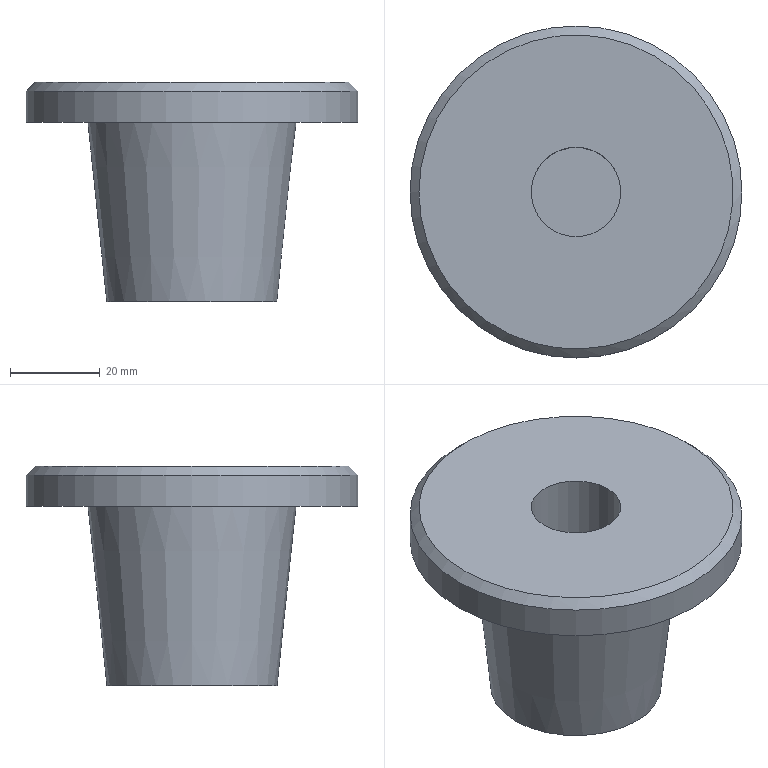Component | NX | CH3404_19_3-6 | 1 solid | 8 faces | box 74 x 74 x 49 mm | volume 82142 mm3 | plane 4 | cylinder 2 | cone 2 | commonest cylinder face diameters 74 x1 20 x1
STEP:
#1=CARTESIAN_POINT('',(0.,0.,0.));
#2=DIRECTION('',(0.,0.,1.));
#3=DIRECTION('',(1.,0.,0.));
#4=AXIS2_PLACEMENT_3D('',#1,#2,#3);
#5=CARTESIAN_POINT('',(-37.,0.,96.55));
#6=VERTEX_POINT('',#5);
#7=CARTESIAN_POINT('',(0.,0.,96.55));
#8=DIRECTION('',(0.,0.,-1.));
#9=DIRECTION('',(-1.,0.,0.));
#10=AXIS2_PLACEMENT_3D('',#7,#8,#9);
#11=CIRCLE('',#10,37.);
#12=CARTESIAN_POINT('',(0.,0.,56.55));
#13=DIRECTION('',(0.,0.,-1.));
#14=DIRECTION('',(-1.,0.,0.));
#15=AXIS2_PLACEMENT_3D('',#12,#13,#14);
#16=CYLINDRICAL_SURFACE('',#15,37.);
#17=CARTESIAN_POINT('',(0.,-40.));
#18=DIRECTION('',(1.,0.));
#19=VECTOR('',#18,1.);
#20=LINE('',#17,#19);
#21=(GEOMETRIC_REPRESENTATION_CONTEXT(2)PARAMETRIC_REPRESENTATION_CONTEXT()REPRESENTATION_CONTEXT('',''));
#22=DEFINITIONAL_REPRESENTATION('',(#20),#21);
#23=PCURVE('',#16,#22);
#24=CARTESIAN_POINT('',(0.,-37.,96.55));
#25=DIRECTION('',(0.,0.,1.));
#26=DIRECTION('',(1.,0.,0.));
#27=AXIS2_PLACEMENT_3D('',#24,#25,#26);
#28=PLANE('',#27);
#29=CARTESIAN_POINT('',(-37.,37.));
#30=CARTESIAN_POINT('',(-37.,101.086));
#31=CARTESIAN_POINT('',(18.5,69.043));
#32=CARTESIAN_POINT('',(74.,37.));
#33=CARTESIAN_POINT('',(18.5,4.957));
#34=CARTESIAN_POINT('',(-37.,-27.086));
#35=CARTESIAN_POINT('',(-37.,37.));
#36=(BOUNDED_CURVE()B_SPLINE_CURVE(2,(#29,#30,#31,#32,#33,#34,#35),.UNSPECIFIED.,.T.,.F.)B_SPLINE_CURVE_WITH_KNOTS((1,2,2,2,2,1),(-2.094,0.,2.094,4.189,6.283,8.378),.UNSPECIFIED.)CURVE()GEOMETRIC_REPRESENTATION_ITEM()RATIONAL_B_SPLINE_CURVE((1.,0.5,1.,0.5,1.,0.5,1.))REPRESENTATION_ITEM(''));
#37=(GEOMETRIC_REPRESENTATION_CONTEXT(2)PARAMETRIC_REPRESENTATION_CONTEXT()REPRESENTATION_CONTEXT('',''));
#38=DEFINITIONAL_REPRESENTATION('',(#36),#37);
#39=PCURVE('',#28,#38);
#40=SURFACE_CURVE('',#11,(#23,#39),.PCURVE_S1.);
#41=EDGE_CURVE('',#6,#6,#40,.T.);
#42=ORIENTED_EDGE('',*,*,#41,.F.);
#43=CARTESIAN_POINT('',(-37.,0.,103.55));
#44=VERTEX_POINT('',#43);
#45=CARTESIAN_POINT('',(-37.,-0.,103.55));
#46=CARTESIAN_POINT('',(-37.,-0.,96.55));
#47=B_SPLINE_CURVE_WITH_KNOTS('',1,(#45,#46),.UNSPECIFIED.,.F.,.F.,(2,2),(-47.,-40.),.PIECEWISE_BEZIER_KNOTS.);
#48=CARTESIAN_POINT('',(0.,0.));
#49=DIRECTION('',(0.,1.));
#50=VECTOR('',#49,1.);
#51=LINE('',#48,#50);
#52=(GEOMETRIC_REPRESENTATION_CONTEXT(2)PARAMETRIC_REPRESENTATION_CONTEXT()REPRESENTATION_CONTEXT('',''));
#53=DEFINITIONAL_REPRESENTATION('',(#51),#52);
#54=PCURVE('',#16,#53);
#55=CARTESIAN_POINT('',(6.283,0.));
#56=DIRECTION('',(0.,1.));
#57=VECTOR('',#56,1.);
#58=LINE('',#55,#57);
#59=(GEOMETRIC_REPRESENTATION_CONTEXT(2)PARAMETRIC_REPRESENTATION_CONTEXT()REPRESENTATION_CONTEXT('',''));
#60=DEFINITIONAL_REPRESENTATION('',(#58),#59);
#61=PCURVE('',#16,#60);
#62=SEAM_CURVE('',#47,(#54,#61),.PCURVE_S1.);
#63=EDGE_CURVE('',#44,#6,#62,.T.);
#64=ORIENTED_EDGE('',*,*,#63,.F.);
#65=CARTESIAN_POINT('',(0.,0.,103.55));
#66=DIRECTION('',(0.,0.,-1.));
#67=DIRECTION('',(-1.,0.,0.));
#68=AXIS2_PLACEMENT_3D('',#65,#66,#67);
#69=CIRCLE('',#68,37.);
#70=CARTESIAN_POINT('',(0.,-47.));
#71=DIRECTION('',(1.,0.));
#72=VECTOR('',#71,1.);
#73=LINE('',#70,#72);
#74=(GEOMETRIC_REPRESENTATION_CONTEXT(2)PARAMETRIC_REPRESENTATION_CONTEXT()REPRESENTATION_CONTEXT('',''));
#75=DEFINITIONAL_REPRESENTATION('',(#73),#74);
#76=PCURVE('',#16,#75);
#77=CARTESIAN_POINT('',(0.,0.,105.55));
#78=DIRECTION('',(0.,0.,-1.));
#79=DIRECTION('',(-1.,0.,0.));
#80=AXIS2_PLACEMENT_3D('',#77,#78,#79);
#81=CONICAL_SURFACE('',#80,35.,0.7854);
#82=CARTESIAN_POINT('',(0.,2.));
#83=DIRECTION('',(1.,0.));
#84=VECTOR('',#83,1.);
#85=LINE('',#82,#84);
#86=(GEOMETRIC_REPRESENTATION_CONTEXT(2)PARAMETRIC_REPRESENTATION_CONTEXT()REPRESENTATION_CONTEXT('',''));
#87=DEFINITIONAL_REPRESENTATION('',(#85),#86);
#88=PCURVE('',#81,#87);
#89=SURFACE_CURVE('',#69,(#76,#88),.PCURVE_S1.);
#90=EDGE_CURVE('',#44,#44,#89,.T.);
#91=ORIENTED_EDGE('',*,*,#90,.T.);
#92=ORIENTED_EDGE('',*,*,#63,.T.);
#93=EDGE_LOOP('',(#42,#64,#91,#92));
#94=FACE_BOUND('',#93,.T.);
#95=ADVANCED_FACE('',(#94),#16,.T.);
#96=CARTESIAN_POINT('',(-23.204,0.,96.55));
#97=VERTEX_POINT('',#96);
#98=CARTESIAN_POINT('',(0.,0.,96.55));
#99=DIRECTION('',(0.,0.,-1.));
#100=DIRECTION('',(-1.,0.,0.));
#101=AXIS2_PLACEMENT_3D('',#98,#99,#100);
#102=CIRCLE('',#101,23.204);
#103=CARTESIAN_POINT('',(-23.204,37.));
#104=CARTESIAN_POINT('',(-23.204,77.191));
#105=CARTESIAN_POINT('',(11.602,57.095));
#106=CARTESIAN_POINT('',(46.408,37.));
#107=CARTESIAN_POINT('',(11.602,16.905));
#108=CARTESIAN_POINT('',(-23.204,-3.191));
#109=CARTESIAN_POINT('',(-23.204,37.));
#110=(BOUNDED_CURVE()B_SPLINE_CURVE(2,(#103,#104,#105,#106,#107,#108,#109),.UNSPECIFIED.,.T.,.F.)B_SPLINE_CURVE_WITH_KNOTS((1,2,2,2,2,1),(-2.094,0.,2.094,4.189,6.283,8.378),.UNSPECIFIED.)CURVE()GEOMETRIC_REPRESENTATION_ITEM()RATIONAL_B_SPLINE_CURVE((1.,0.5,1.,0.5,1.,0.5,1.))REPRESENTATION_ITEM(''));
#111=(GEOMETRIC_REPRESENTATION_CONTEXT(2)PARAMETRIC_REPRESENTATION_CONTEXT()REPRESENTATION_CONTEXT('',''));
#112=DEFINITIONAL_REPRESENTATION('',(#110),#111);
#113=PCURVE('',#28,#112);
#114=CARTESIAN_POINT('',(0.,0.,96.55));
#115=DIRECTION('',(0.,0.,1.));
#116=DIRECTION('',(1.,0.,0.));
#117=AXIS2_PLACEMENT_3D('',#114,#115,#116);
#118=CONICAL_SURFACE('',#117,23.204,0.1047);
#119=CARTESIAN_POINT('',(9.425,0.));
#120=DIRECTION('',(-1.,0.));
#121=VECTOR('',#120,1.);
#122=LINE('',#119,#121);
#123=(GEOMETRIC_REPRESENTATION_CONTEXT(2)PARAMETRIC_REPRESENTATION_CONTEXT()REPRESENTATION_CONTEXT('',''));
#124=DEFINITIONAL_REPRESENTATION('',(#122),#123);
#125=PCURVE('',#118,#124);
#126=SURFACE_CURVE('',#102,(#113,#125),.PCURVE_S1.);
#127=EDGE_CURVE('',#97,#97,#126,.T.);
#128=ORIENTED_EDGE('',*,*,#127,.F.);
#129=EDGE_LOOP('',(#128));
#130=FACE_BOUND('',#129,.T.);
#131=ORIENTED_EDGE('',*,*,#41,.T.);
#132=EDGE_LOOP('',(#131));
#133=FACE_BOUND('',#132,.T.);
#134=ADVANCED_FACE('',(#130,#133),#28,.F.);
#135=CARTESIAN_POINT('',(-19.,0.,56.55));
#136=VERTEX_POINT('',#135);
#137=CARTESIAN_POINT('',(0.,0.,56.55));
#138=DIRECTION('',(0.,0.,-1.));
#139=DIRECTION('',(-1.,0.,0.));
#140=AXIS2_PLACEMENT_3D('',#137,#138,#139);
#141=CIRCLE('',#140,19.);
#142=CARTESIAN_POINT('',(9.425,-40.));
#143=DIRECTION('',(-1.,0.));
#144=VECTOR('',#143,1.);
#145=LINE('',#142,#144);
#146=(GEOMETRIC_REPRESENTATION_CONTEXT(2)PARAMETRIC_REPRESENTATION_CONTEXT()REPRESENTATION_CONTEXT('',''));
#147=DEFINITIONAL_REPRESENTATION('',(#145),#146);
#148=PCURVE('',#118,#147);
#149=CARTESIAN_POINT('',(0.,-19.,56.55));
#150=DIRECTION('',(0.,0.,1.));
#151=DIRECTION('',(1.,0.,0.));
#152=AXIS2_PLACEMENT_3D('',#149,#150,#151);
#153=PLANE('',#152);
#154=CARTESIAN_POINT('',(-19.,19.));
#155=CARTESIAN_POINT('',(-19.,51.909));
#156=CARTESIAN_POINT('',(9.5,35.454));
#157=CARTESIAN_POINT('',(38.,19.));
#158=CARTESIAN_POINT('',(9.5,2.546));
#159=CARTESIAN_POINT('',(-19.,-13.909));
#160=CARTESIAN_POINT('',(-19.,19.));
#161=(BOUNDED_CURVE()B_SPLINE_CURVE(2,(#154,#155,#156,#157,#158,#159,#160),.UNSPECIFIED.,.T.,.F.)B_SPLINE_CURVE_WITH_KNOTS((1,2,2,2,2,1),(-2.094,0.,2.094,4.189,6.283,8.378),.UNSPECIFIED.)CURVE()GEOMETRIC_REPRESENTATION_ITEM()RATIONAL_B_SPLINE_CURVE((1.,0.5,1.,0.5,1.,0.5,1.))REPRESENTATION_ITEM(''));
#162=(GEOMETRIC_REPRESENTATION_CONTEXT(2)PARAMETRIC_REPRESENTATION_CONTEXT()REPRESENTATION_CONTEXT('',''));
#163=DEFINITIONAL_REPRESENTATION('',(#161),#162);
#164=PCURVE('',#153,#163);
#165=SURFACE_CURVE('',#141,(#148,#164),.PCURVE_S1.);
#166=EDGE_CURVE('',#136,#136,#165,.T.);
#167=ORIENTED_EDGE('',*,*,#166,.F.);
#168=CARTESIAN_POINT('',(-19.,0.,56.55));
#169=CARTESIAN_POINT('',(-23.204,0.,96.55));
#170=B_SPLINE_CURVE_WITH_KNOTS('',1,(#168,#169),.UNSPECIFIED.,.F.,.F.,(2,2),(-40.22,0.),.PIECEWISE_BEZIER_KNOTS.);
#171=CARTESIAN_POINT('',(9.425,0.));
#172=DIRECTION('',(0.,1.));
#173=VECTOR('',#172,1.);
#174=LINE('',#171,#173);
#175=(GEOMETRIC_REPRESENTATION_CONTEXT(2)PARAMETRIC_REPRESENTATION_CONTEXT()REPRESENTATION_CONTEXT('',''));
#176=DEFINITIONAL_REPRESENTATION('',(#174),#175);
#177=PCURVE('',#118,#176);
#178=CARTESIAN_POINT('',(3.142,0.));
#179=DIRECTION('',(0.,1.));
#180=VECTOR('',#179,1.);
#181=LINE('',#178,#180);
#182=(GEOMETRIC_REPRESENTATION_CONTEXT(2)PARAMETRIC_REPRESENTATION_CONTEXT()REPRESENTATION_CONTEXT('',''));
#183=DEFINITIONAL_REPRESENTATION('',(#181),#182);
#184=PCURVE('',#118,#183);
#185=SEAM_CURVE('',#170,(#177,#184),.PCURVE_S1.);
#186=EDGE_CURVE('',#136,#97,#185,.T.);
#187=ORIENTED_EDGE('',*,*,#186,.T.);
#188=ORIENTED_EDGE('',*,*,#127,.T.);
#189=ORIENTED_EDGE('',*,*,#186,.F.);
#190=EDGE_LOOP('',(#167,#187,#188,#189));
#191=FACE_BOUND('',#190,.T.);
#192=ADVANCED_FACE('',(#191),#118,.T.);
#193=ORIENTED_EDGE('',*,*,#166,.T.);
#194=EDGE_LOOP('',(#193));
#195=FACE_BOUND('',#194,.T.);
#196=ADVANCED_FACE('',(#195),#153,.F.);
#197=CARTESIAN_POINT('',(-10.,0.,66.55));
#198=VERTEX_POINT('',#197);
#199=CARTESIAN_POINT('',(0.,0.,66.55));
#200=DIRECTION('',(0.,0.,-1.));
#201=DIRECTION('',(-1.,0.,0.));
#202=AXIS2_PLACEMENT_3D('',#199,#200,#201);
#203=CIRCLE('',#202,10.);
#204=CARTESIAN_POINT('',(0.,0.,66.55));
#205=DIRECTION('',(0.,0.,-1.));
#206=DIRECTION('',(-1.,0.,0.));
#207=AXIS2_PLACEMENT_3D('',#204,#205,#206);
#208=PLANE('',#207);
#209=CARTESIAN_POINT('',(0.,0.));
#210=DIRECTION('',(1.,0.));
#211=AXIS2_PLACEMENT_2D('',#209,#210);
#212=CIRCLE('',#211,10.);
#213=(GEOMETRIC_REPRESENTATION_CONTEXT(2)PARAMETRIC_REPRESENTATION_CONTEXT()REPRESENTATION_CONTEXT('',''));
#214=DEFINITIONAL_REPRESENTATION('',(#212),#213);
#215=PCURVE('',#208,#214);
#216=CARTESIAN_POINT('',(0.,0.,56.55));
#217=DIRECTION('',(0.,0.,-1.));
#218=DIRECTION('',(-1.,0.,0.));
#219=AXIS2_PLACEMENT_3D('',#216,#217,#218);
#220=CYLINDRICAL_SURFACE('',#219,10.);
#221=CARTESIAN_POINT('',(0.,-10.));
#222=DIRECTION('',(1.,0.));
#223=VECTOR('',#222,1.);
#224=LINE('',#221,#223);
#225=(GEOMETRIC_REPRESENTATION_CONTEXT(2)PARAMETRIC_REPRESENTATION_CONTEXT()REPRESENTATION_CONTEXT('',''));
#226=DEFINITIONAL_REPRESENTATION('',(#224),#225);
#227=PCURVE('',#220,#226);
#228=SURFACE_CURVE('',#203,(#215,#227),.PCURVE_S1.);
#229=EDGE_CURVE('',#198,#198,#228,.T.);
#230=ORIENTED_EDGE('',*,*,#229,.F.);
#231=EDGE_LOOP('',(#230));
#232=FACE_BOUND('',#231,.T.);
#233=ADVANCED_FACE('',(#232),#208,.F.);
#234=CARTESIAN_POINT('',(-10.,0.,105.55));
#235=VERTEX_POINT('',#234);
#236=CARTESIAN_POINT('',(0.,0.,105.55));
#237=DIRECTION('',(0.,0.,-1.));
#238=DIRECTION('',(-1.,0.,0.));
#239=AXIS2_PLACEMENT_3D('',#236,#237,#238);
#240=CIRCLE('',#239,10.);
#241=CARTESIAN_POINT('',(0.,-49.));
#242=DIRECTION('',(1.,0.));
#243=VECTOR('',#242,1.);
#244=LINE('',#241,#243);
#245=(GEOMETRIC_REPRESENTATION_CONTEXT(2)PARAMETRIC_REPRESENTATION_CONTEXT()REPRESENTATION_CONTEXT('',''));
#246=DEFINITIONAL_REPRESENTATION('',(#244),#245);
#247=PCURVE('',#220,#246);
#248=CARTESIAN_POINT('',(0.,-10.,105.55));
#249=DIRECTION('',(0.,0.,-1.));
#250=DIRECTION('',(-1.,0.,0.));
#251=AXIS2_PLACEMENT_3D('',#248,#249,#250);
#252=PLANE('',#251);
#253=CARTESIAN_POINT('',(0.,10.));
#254=DIRECTION('',(1.,0.));
#255=AXIS2_PLACEMENT_2D('',#253,#254);
#256=CIRCLE('',#255,10.);
#257=(GEOMETRIC_REPRESENTATION_CONTEXT(2)PARAMETRIC_REPRESENTATION_CONTEXT()REPRESENTATION_CONTEXT('',''));
#258=DEFINITIONAL_REPRESENTATION('',(#256),#257);
#259=PCURVE('',#252,#258);
#260=SURFACE_CURVE('',#240,(#247,#259),.PCURVE_S1.);
#261=EDGE_CURVE('',#235,#235,#260,.T.);
#262=ORIENTED_EDGE('',*,*,#261,.T.);
#263=CARTESIAN_POINT('',(-10.,0.,105.55));
#264=CARTESIAN_POINT('',(-10.,0.,66.55));
#265=B_SPLINE_CURVE_WITH_KNOTS('',1,(#263,#264),.UNSPECIFIED.,.F.,.F.,(2,2),(-49.,-10.),.PIECEWISE_BEZIER_KNOTS.);
#266=CARTESIAN_POINT('',(6.283,0.));
#267=DIRECTION('',(0.,1.));
#268=VECTOR('',#267,1.);
#269=LINE('',#266,#268);
#270=(GEOMETRIC_REPRESENTATION_CONTEXT(2)PARAMETRIC_REPRESENTATION_CONTEXT()REPRESENTATION_CONTEXT('',''));
#271=DEFINITIONAL_REPRESENTATION('',(#269),#270);
#272=PCURVE('',#220,#271);
#273=CARTESIAN_POINT('',(0.,0.));
#274=DIRECTION('',(0.,1.));
#275=VECTOR('',#274,1.);
#276=LINE('',#273,#275);
#277=(GEOMETRIC_REPRESENTATION_CONTEXT(2)PARAMETRIC_REPRESENTATION_CONTEXT()REPRESENTATION_CONTEXT('',''));
#278=DEFINITIONAL_REPRESENTATION('',(#276),#277);
#279=PCURVE('',#220,#278);
#280=SEAM_CURVE('',#265,(#272,#279),.PCURVE_S1.);
#281=EDGE_CURVE('',#235,#198,#280,.T.);
#282=ORIENTED_EDGE('',*,*,#281,.T.);
#283=ORIENTED_EDGE('',*,*,#229,.F.);
#284=ORIENTED_EDGE('',*,*,#281,.F.);
#285=EDGE_LOOP('',(#262,#282,#283,#284));
#286=FACE_BOUND('',#285,.F.);
#287=ADVANCED_FACE('',(#286),#220,.F.);
#288=CARTESIAN_POINT('',(-35.,0.,105.55));
#289=VERTEX_POINT('',#288);
#290=CARTESIAN_POINT('',(0.,0.,105.55));
#291=DIRECTION('',(0.,0.,-1.));
#292=DIRECTION('',(-1.,0.,0.));
#293=AXIS2_PLACEMENT_3D('',#290,#291,#292);
#294=CIRCLE('',#293,35.);
#295=CARTESIAN_POINT('',(0.,10.));
#296=DIRECTION('',(1.,0.));
#297=AXIS2_PLACEMENT_2D('',#295,#296);
#298=CIRCLE('',#297,35.);
#299=(GEOMETRIC_REPRESENTATION_CONTEXT(2)PARAMETRIC_REPRESENTATION_CONTEXT()REPRESENTATION_CONTEXT('',''));
#300=DEFINITIONAL_REPRESENTATION('',(#298),#299);
#301=PCURVE('',#252,#300);
#302=CARTESIAN_POINT('',(0.,0.));
#303=DIRECTION('',(1.,0.));
#304=VECTOR('',#303,1.);
#305=LINE('',#302,#304);
#306=(GEOMETRIC_REPRESENTATION_CONTEXT(2)PARAMETRIC_REPRESENTATION_CONTEXT()REPRESENTATION_CONTEXT('',''));
#307=DEFINITIONAL_REPRESENTATION('',(#305),#306);
#308=PCURVE('',#81,#307);
#309=SURFACE_CURVE('',#294,(#301,#308),.PCURVE_S1.);
#310=EDGE_CURVE('',#289,#289,#309,.T.);
#311=ORIENTED_EDGE('',*,*,#310,.F.);
#312=EDGE_LOOP('',(#311));
#313=FACE_BOUND('',#312,.T.);
#314=ORIENTED_EDGE('',*,*,#261,.T.);
#315=EDGE_LOOP('',(#314));
#316=FACE_BOUND('',#315,.T.);
#317=ADVANCED_FACE('',(#313,#316),#252,.F.);
#318=ORIENTED_EDGE('',*,*,#90,.F.);
#319=CARTESIAN_POINT('',(-35.,-0.,105.55));
#320=CARTESIAN_POINT('',(-37.,-0.,103.55));
#321=B_SPLINE_CURVE_WITH_KNOTS('',1,(#319,#320),.UNSPECIFIED.,.F.,.F.,(2,2),(0.,2.828),.PIECEWISE_BEZIER_KNOTS.);
#322=CARTESIAN_POINT('',(0.,0.));
#323=DIRECTION('',(0.,1.));
#324=VECTOR('',#323,1.);
#325=LINE('',#322,#324);
#326=(GEOMETRIC_REPRESENTATION_CONTEXT(2)PARAMETRIC_REPRESENTATION_CONTEXT()REPRESENTATION_CONTEXT('',''));
#327=DEFINITIONAL_REPRESENTATION('',(#325),#326);
#328=PCURVE('',#81,#327);
#329=CARTESIAN_POINT('',(6.283,0.));
#330=DIRECTION('',(0.,1.));
#331=VECTOR('',#330,1.);
#332=LINE('',#329,#331);
#333=(GEOMETRIC_REPRESENTATION_CONTEXT(2)PARAMETRIC_REPRESENTATION_CONTEXT()REPRESENTATION_CONTEXT('',''));
#334=DEFINITIONAL_REPRESENTATION('',(#332),#333);
#335=PCURVE('',#81,#334);
#336=SEAM_CURVE('',#321,(#328,#335),.PCURVE_S1.);
#337=EDGE_CURVE('',#289,#44,#336,.T.);
#338=ORIENTED_EDGE('',*,*,#337,.F.);
#339=ORIENTED_EDGE('',*,*,#310,.T.);
#340=ORIENTED_EDGE('',*,*,#337,.T.);
#341=EDGE_LOOP('',(#318,#338,#339,#340));
#342=FACE_BOUND('',#341,.T.);
#343=ADVANCED_FACE('',(#342),#81,.T.);
#344=CLOSED_SHELL('',(#95,#134,#192,#196,#233,#287,#317,#343));
#345=MANIFOLD_SOLID_BREP('',#344);
#346=(LENGTH_UNIT()NAMED_UNIT(*)SI_UNIT(.MILLI.,.METRE.));
#347=UNCERTAINTY_MEASURE_WITH_UNIT(LENGTH_MEASURE(0.00001),#346,'','');
#348=(NAMED_UNIT(*)PLANE_ANGLE_UNIT()SI_UNIT($,.RADIAN.));
#349=(NAMED_UNIT(*)SI_UNIT($,.STERADIAN.)SOLID_ANGLE_UNIT());
#350=(GEOMETRIC_REPRESENTATION_CONTEXT(3)GLOBAL_UNCERTAINTY_ASSIGNED_CONTEXT((#347))GLOBAL_UNIT_ASSIGNED_CONTEXT((#346,#348,#349))REPRESENTATION_CONTEXT('',''));
#351=ADVANCED_BREP_SHAPE_REPRESENTATION('',(#4,#345),#350);